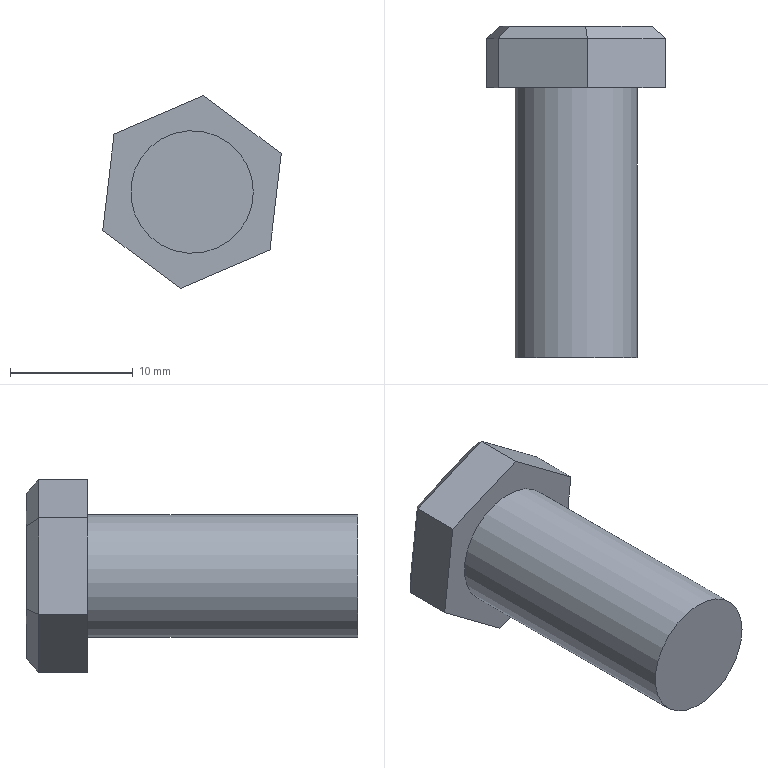Component | NX | LOC_PIN_2 | 1 solid | 16 faces | box 14.55 x 27 x 15.73 mm | volume 2520 mm3 | plane 15 | cylinder 1 | commonest cylinder face diameters 10 x1
STEP:
#1=CARTESIAN_POINT('',(0.,0.,0.));
#2=DIRECTION('',(0.,0.,1.));
#3=DIRECTION('',(1.,0.,0.));
#4=AXIS2_PLACEMENT_3D('',#1,#2,#3);
#5=CARTESIAN_POINT('',(68.825,100.796,50.));
#6=VERTEX_POINT('',#5);
#7=CARTESIAN_POINT('',(63.825,100.796,50.));
#8=DIRECTION('',(0.,-1.,0.));
#9=DIRECTION('',(1.,0.,0.));
#10=AXIS2_PLACEMENT_3D('',#7,#8,#9);
#11=CIRCLE('',#10,5.);
#12=CARTESIAN_POINT('',(63.825,100.796,50.));
#13=DIRECTION('',(0.,-1.,0.));
#14=DIRECTION('',(-1.,0.,0.));
#15=AXIS2_PLACEMENT_3D('',#12,#13,#14);
#16=CYLINDRICAL_SURFACE('',#15,5.);
#17=CARTESIAN_POINT('',(3.142,0.));
#18=DIRECTION('',(1.,0.));
#19=VECTOR('',#18,1.);
#20=LINE('',#17,#19);
#21=(GEOMETRIC_REPRESENTATION_CONTEXT(2)PARAMETRIC_REPRESENTATION_CONTEXT()REPRESENTATION_CONTEXT('',''));
#22=DEFINITIONAL_REPRESENTATION('',(#20),#21);
#23=PCURVE('',#16,#22);
#24=CARTESIAN_POINT('',(63.825,100.796,50.));
#25=DIRECTION('',(0.,-1.,0.));
#26=DIRECTION('',(-1.,0.,0.));
#27=AXIS2_PLACEMENT_3D('',#24,#25,#26);
#28=PLANE('',#27);
#29=CARTESIAN_POINT('',(0.,0.));
#30=DIRECTION('',(-1.,0.));
#31=AXIS2_PLACEMENT_2D('',#29,#30);
#32=CIRCLE('',#31,5.);
#33=(GEOMETRIC_REPRESENTATION_CONTEXT(2)PARAMETRIC_REPRESENTATION_CONTEXT()REPRESENTATION_CONTEXT('',''));
#34=DEFINITIONAL_REPRESENTATION('',(#32),#33);
#35=PCURVE('',#28,#34);
#36=SURFACE_CURVE('',#11,(#23,#35),.PCURVE_S1.);
#37=EDGE_CURVE('',#6,#6,#36,.T.);
#38=ORIENTED_EDGE('',*,*,#37,.T.);
#39=CARTESIAN_POINT('',(68.825,78.796,50.));
#40=VERTEX_POINT('',#39);
#41=CARTESIAN_POINT('',(68.825,100.796,50.));
#42=CARTESIAN_POINT('',(68.825,78.796,50.));
#43=B_SPLINE_CURVE_WITH_KNOTS('',1,(#41,#42),.UNSPECIFIED.,.F.,.F.,(2,2),(0.,22.),.PIECEWISE_BEZIER_KNOTS.);
#44=CARTESIAN_POINT('',(9.425,0.));
#45=DIRECTION('',(0.,1.));
#46=VECTOR('',#45,1.);
#47=LINE('',#44,#46);
#48=(GEOMETRIC_REPRESENTATION_CONTEXT(2)PARAMETRIC_REPRESENTATION_CONTEXT()REPRESENTATION_CONTEXT('',''));
#49=DEFINITIONAL_REPRESENTATION('',(#47),#48);
#50=PCURVE('',#16,#49);
#51=CARTESIAN_POINT('',(3.142,0.));
#52=DIRECTION('',(0.,1.));
#53=VECTOR('',#52,1.);
#54=LINE('',#51,#53);
#55=(GEOMETRIC_REPRESENTATION_CONTEXT(2)PARAMETRIC_REPRESENTATION_CONTEXT()REPRESENTATION_CONTEXT('',''));
#56=DEFINITIONAL_REPRESENTATION('',(#54),#55);
#57=PCURVE('',#16,#56);
#58=SEAM_CURVE('',#43,(#50,#57),.PCURVE_S1.);
#59=EDGE_CURVE('',#6,#40,#58,.T.);
#60=ORIENTED_EDGE('',*,*,#59,.T.);
#61=CARTESIAN_POINT('',(63.825,78.796,50.));
#62=DIRECTION('',(0.,-1.,0.));
#63=DIRECTION('',(1.,0.,0.));
#64=AXIS2_PLACEMENT_3D('',#61,#62,#63);
#65=CIRCLE('',#64,5.);
#66=CARTESIAN_POINT('',(3.142,22.));
#67=DIRECTION('',(1.,0.));
#68=VECTOR('',#67,1.);
#69=LINE('',#66,#68);
#70=(GEOMETRIC_REPRESENTATION_CONTEXT(2)PARAMETRIC_REPRESENTATION_CONTEXT()REPRESENTATION_CONTEXT('',''));
#71=DEFINITIONAL_REPRESENTATION('',(#69),#70);
#72=PCURVE('',#16,#71);
#73=CARTESIAN_POINT('',(63.825,78.796,50.));
#74=DIRECTION('',(0.,-1.,0.));
#75=DIRECTION('',(-1.,0.,0.));
#76=AXIS2_PLACEMENT_3D('',#73,#74,#75);
#77=PLANE('',#76);
#78=CARTESIAN_POINT('',(0.,0.));
#79=DIRECTION('',(-1.,0.));
#80=AXIS2_PLACEMENT_2D('',#78,#79);
#81=CIRCLE('',#80,5.);
#82=(GEOMETRIC_REPRESENTATION_CONTEXT(2)PARAMETRIC_REPRESENTATION_CONTEXT()REPRESENTATION_CONTEXT('',''));
#83=DEFINITIONAL_REPRESENTATION('',(#81),#82);
#84=PCURVE('',#77,#83);
#85=SURFACE_CURVE('',#65,(#72,#84),.PCURVE_S1.);
#86=EDGE_CURVE('',#40,#40,#85,.T.);
#87=ORIENTED_EDGE('',*,*,#86,.F.);
#88=ORIENTED_EDGE('',*,*,#59,.F.);
#89=EDGE_LOOP('',(#38,#60,#87,#88));
#90=FACE_BOUND('',#89,.T.);
#91=ADVANCED_FACE('',(#90),#16,.T.);
#92=ORIENTED_EDGE('',*,*,#86,.T.);
#93=EDGE_LOOP('',(#92));
#94=FACE_BOUND('',#93,.T.);
#95=ADVANCED_FACE('',(#94),#77,.T.);
#96=CARTESIAN_POINT('',(56.548,104.796,46.869));
#97=VERTEX_POINT('',#96);
#98=CARTESIAN_POINT('',(56.548,100.796,46.869));
#99=VERTEX_POINT('',#98);
#100=CARTESIAN_POINT('',(56.548,105.796,46.869));
#101=DIRECTION('',(0.,-1.,0.));
#102=VECTOR('',#101,1.);
#103=LINE('',#100,#102);
#104=CARTESIAN_POINT('',(56.548,105.796,46.869));
#105=DIRECTION('',(-0.5979,0.,-0.8016));
#106=DIRECTION('',(-0.8016,0.,0.5979));
#107=AXIS2_PLACEMENT_3D('',#104,#105,#106);
#108=PLANE('',#107);
#109=CARTESIAN_POINT('',(0.,0.));
#110=DIRECTION('',(0.,-1.));
#111=VECTOR('',#110,1.);
#112=LINE('',#109,#111);
#113=(GEOMETRIC_REPRESENTATION_CONTEXT(2)PARAMETRIC_REPRESENTATION_CONTEXT()REPRESENTATION_CONTEXT('',''));
#114=DEFINITIONAL_REPRESENTATION('',(#112),#113);
#115=PCURVE('',#108,#114);
#116=CARTESIAN_POINT('',(57.475,105.796,54.736));
#117=DIRECTION('',(-0.9931,0.,0.117));
#118=DIRECTION('',(0.117,0.,0.9931));
#119=AXIS2_PLACEMENT_3D('',#116,#117,#118);
#120=PLANE('',#119);
#121=CARTESIAN_POINT('',(-7.922,0.));
#122=DIRECTION('',(0.,-1.));
#123=VECTOR('',#122,1.);
#124=LINE('',#121,#123);
#125=(GEOMETRIC_REPRESENTATION_CONTEXT(2)PARAMETRIC_REPRESENTATION_CONTEXT()REPRESENTATION_CONTEXT('',''));
#126=DEFINITIONAL_REPRESENTATION('',(#124),#125);
#127=PCURVE('',#120,#126);
#128=SURFACE_CURVE('',#103,(#115,#127),.PCURVE_S1.);
#129=EDGE_CURVE('',#97,#99,#128,.T.);
#130=ORIENTED_EDGE('',*,*,#129,.F.);
#131=CARTESIAN_POINT('',(62.898,104.796,42.133));
#132=VERTEX_POINT('',#131);
#133=CARTESIAN_POINT('',(62.898,104.796,42.133));
#134=DIRECTION('',(0.8016,0.,-0.5979));
#135=VECTOR('',#134,1.);
#136=LINE('',#133,#135);
#137=CARTESIAN_POINT('',(-7.922,-1.));
#138=DIRECTION('',(-1.,0.));
#139=VECTOR('',#138,1.);
#140=LINE('',#137,#139);
#141=(GEOMETRIC_REPRESENTATION_CONTEXT(2)PARAMETRIC_REPRESENTATION_CONTEXT()REPRESENTATION_CONTEXT('',''));
#142=DEFINITIONAL_REPRESENTATION('',(#140),#141);
#143=PCURVE('',#108,#142);
#144=CARTESIAN_POINT('',(56.548,104.796,46.869));
#145=DIRECTION('',(-0.4228,0.7071,-0.5668));
#146=DIRECTION('',(-0.8016,0.,0.5979));
#147=AXIS2_PLACEMENT_3D('',#144,#145,#146);
#148=PLANE('',#147);
#149=CARTESIAN_POINT('',(-7.922,-0.));
#150=DIRECTION('',(-1.,0.));
#151=VECTOR('',#150,1.);
#152=LINE('',#149,#151);
#153=(GEOMETRIC_REPRESENTATION_CONTEXT(2)PARAMETRIC_REPRESENTATION_CONTEXT()REPRESENTATION_CONTEXT('',''));
#154=DEFINITIONAL_REPRESENTATION('',(#152),#153);
#155=PCURVE('',#148,#154);
#156=SURFACE_CURVE('',#136,(#143,#155),.PCURVE_S1.);
#157=EDGE_CURVE('',#97,#132,#156,.T.);
#158=ORIENTED_EDGE('',*,*,#157,.T.);
#159=CARTESIAN_POINT('',(62.898,100.796,42.133));
#160=VERTEX_POINT('',#159);
#161=CARTESIAN_POINT('',(62.898,105.796,42.133));
#162=DIRECTION('',(0.,-1.,0.));
#163=VECTOR('',#162,1.);
#164=LINE('',#161,#163);
#165=CARTESIAN_POINT('',(-7.922,0.));
#166=DIRECTION('',(0.,-1.));
#167=VECTOR('',#166,1.);
#168=LINE('',#165,#167);
#169=(GEOMETRIC_REPRESENTATION_CONTEXT(2)PARAMETRIC_REPRESENTATION_CONTEXT()REPRESENTATION_CONTEXT('',''));
#170=DEFINITIONAL_REPRESENTATION('',(#168),#169);
#171=PCURVE('',#108,#170);
#172=CARTESIAN_POINT('',(62.898,105.796,42.133));
#173=DIRECTION('',(0.3953,0.,-0.9186));
#174=DIRECTION('',(-0.9186,0.,-0.3953));
#175=AXIS2_PLACEMENT_3D('',#172,#173,#174);
#176=PLANE('',#175);
#177=CARTESIAN_POINT('',(0.,0.));
#178=DIRECTION('',(0.,-1.));
#179=VECTOR('',#178,1.);
#180=LINE('',#177,#179);
#181=(GEOMETRIC_REPRESENTATION_CONTEXT(2)PARAMETRIC_REPRESENTATION_CONTEXT()REPRESENTATION_CONTEXT('',''));
#182=DEFINITIONAL_REPRESENTATION('',(#180),#181);
#183=PCURVE('',#176,#182);
#184=SURFACE_CURVE('',#164,(#171,#183),.PCURVE_S1.);
#185=EDGE_CURVE('',#132,#160,#184,.T.);
#186=ORIENTED_EDGE('',*,*,#185,.T.);
#187=CARTESIAN_POINT('',(56.548,100.796,46.869));
#188=DIRECTION('',(0.8016,0.,-0.5979));
#189=VECTOR('',#188,1.);
#190=LINE('',#187,#189);
#191=CARTESIAN_POINT('',(0.,-5.));
#192=DIRECTION('',(-1.,0.));
#193=VECTOR('',#192,1.);
#194=LINE('',#191,#193);
#195=(GEOMETRIC_REPRESENTATION_CONTEXT(2)PARAMETRIC_REPRESENTATION_CONTEXT()REPRESENTATION_CONTEXT('',''));
#196=DEFINITIONAL_REPRESENTATION('',(#194),#195);
#197=PCURVE('',#108,#196);
#198=CARTESIAN_POINT('',(7.277,3.131));
#199=DIRECTION('',(-0.8016,0.5979));
#200=VECTOR('',#199,1.);
#201=LINE('',#198,#200);
#202=(GEOMETRIC_REPRESENTATION_CONTEXT(2)PARAMETRIC_REPRESENTATION_CONTEXT()REPRESENTATION_CONTEXT('',''));
#203=DEFINITIONAL_REPRESENTATION('',(#201),#202);
#204=PCURVE('',#28,#203);
#205=SURFACE_CURVE('',#190,(#197,#204),.PCURVE_S1.);
#206=EDGE_CURVE('',#99,#160,#205,.T.);
#207=ORIENTED_EDGE('',*,*,#206,.F.);
#208=EDGE_LOOP('',(#130,#158,#186,#207));
#209=FACE_BOUND('',#208,.T.);
#210=ADVANCED_FACE('',(#209),#108,.T.);
#211=ORIENTED_EDGE('',*,*,#185,.F.);
#212=CARTESIAN_POINT('',(70.175,104.796,45.264));
#213=VERTEX_POINT('',#212);
#214=CARTESIAN_POINT('',(70.175,104.796,45.264));
#215=DIRECTION('',(0.9186,0.,0.3953));
#216=VECTOR('',#215,1.);
#217=LINE('',#214,#216);
#218=CARTESIAN_POINT('',(-7.922,-1.));
#219=DIRECTION('',(-1.,0.));
#220=VECTOR('',#219,1.);
#221=LINE('',#218,#220);
#222=(GEOMETRIC_REPRESENTATION_CONTEXT(2)PARAMETRIC_REPRESENTATION_CONTEXT()REPRESENTATION_CONTEXT('',''));
#223=DEFINITIONAL_REPRESENTATION('',(#221),#222);
#224=PCURVE('',#176,#223);
#225=CARTESIAN_POINT('',(62.898,104.796,42.133));
#226=DIRECTION('',(0.2795,0.7071,-0.6495));
#227=DIRECTION('',(-0.9186,0.,-0.3953));
#228=AXIS2_PLACEMENT_3D('',#225,#226,#227);
#229=PLANE('',#228);
#230=CARTESIAN_POINT('',(-7.922,-0.));
#231=DIRECTION('',(-1.,0.));
#232=VECTOR('',#231,1.);
#233=LINE('',#230,#232);
#234=(GEOMETRIC_REPRESENTATION_CONTEXT(2)PARAMETRIC_REPRESENTATION_CONTEXT()REPRESENTATION_CONTEXT('',''));
#235=DEFINITIONAL_REPRESENTATION('',(#233),#234);
#236=PCURVE('',#229,#235);
#237=SURFACE_CURVE('',#217,(#224,#236),.PCURVE_S1.);
#238=EDGE_CURVE('',#132,#213,#237,.T.);
#239=ORIENTED_EDGE('',*,*,#238,.T.);
#240=CARTESIAN_POINT('',(70.175,100.796,45.264));
#241=VERTEX_POINT('',#240);
#242=CARTESIAN_POINT('',(70.175,105.796,45.264));
#243=DIRECTION('',(0.,-1.,0.));
#244=VECTOR('',#243,1.);
#245=LINE('',#242,#244);
#246=CARTESIAN_POINT('',(-7.922,0.));
#247=DIRECTION('',(0.,-1.));
#248=VECTOR('',#247,1.);
#249=LINE('',#246,#248);
#250=(GEOMETRIC_REPRESENTATION_CONTEXT(2)PARAMETRIC_REPRESENTATION_CONTEXT()REPRESENTATION_CONTEXT('',''));
#251=DEFINITIONAL_REPRESENTATION('',(#249),#250);
#252=PCURVE('',#176,#251);
#253=CARTESIAN_POINT('',(70.175,105.796,45.264));
#254=DIRECTION('',(0.9931,0.,-0.117));
#255=DIRECTION('',(-0.117,0.,-0.9931));
#256=AXIS2_PLACEMENT_3D('',#253,#254,#255);
#257=PLANE('',#256);
#258=CARTESIAN_POINT('',(0.,0.));
#259=DIRECTION('',(0.,-1.));
#260=VECTOR('',#259,1.);
#261=LINE('',#258,#260);
#262=(GEOMETRIC_REPRESENTATION_CONTEXT(2)PARAMETRIC_REPRESENTATION_CONTEXT()REPRESENTATION_CONTEXT('',''));
#263=DEFINITIONAL_REPRESENTATION('',(#261),#262);
#264=PCURVE('',#257,#263);
#265=SURFACE_CURVE('',#245,(#252,#264),.PCURVE_S1.);
#266=EDGE_CURVE('',#213,#241,#265,.T.);
#267=ORIENTED_EDGE('',*,*,#266,.T.);
#268=CARTESIAN_POINT('',(62.898,100.796,42.133));
#269=DIRECTION('',(0.9186,0.,0.3953));
#270=VECTOR('',#269,1.);
#271=LINE('',#268,#270);
#272=CARTESIAN_POINT('',(0.,-5.));
#273=DIRECTION('',(-1.,0.));
#274=VECTOR('',#273,1.);
#275=LINE('',#272,#274);
#276=(GEOMETRIC_REPRESENTATION_CONTEXT(2)PARAMETRIC_REPRESENTATION_CONTEXT()REPRESENTATION_CONTEXT('',''));
#277=DEFINITIONAL_REPRESENTATION('',(#275),#276);
#278=PCURVE('',#176,#277);
#279=CARTESIAN_POINT('',(0.9266,7.867));
#280=DIRECTION('',(-0.9186,-0.3953));
#281=VECTOR('',#280,1.);
#282=LINE('',#279,#281);
#283=(GEOMETRIC_REPRESENTATION_CONTEXT(2)PARAMETRIC_REPRESENTATION_CONTEXT()REPRESENTATION_CONTEXT('',''));
#284=DEFINITIONAL_REPRESENTATION('',(#282),#283);
#285=PCURVE('',#28,#284);
#286=SURFACE_CURVE('',#271,(#278,#285),.PCURVE_S1.);
#287=EDGE_CURVE('',#160,#241,#286,.T.);
#288=ORIENTED_EDGE('',*,*,#287,.F.);
#289=EDGE_LOOP('',(#211,#239,#267,#288));
#290=FACE_BOUND('',#289,.T.);
#291=ADVANCED_FACE('',(#290),#176,.T.);
#292=ORIENTED_EDGE('',*,*,#266,.F.);
#293=CARTESIAN_POINT('',(71.101,104.796,53.131));
#294=VERTEX_POINT('',#293);
#295=CARTESIAN_POINT('',(71.101,104.796,53.131));
#296=DIRECTION('',(0.117,0.,0.9931));
#297=VECTOR('',#296,1.);
#298=LINE('',#295,#297);
#299=CARTESIAN_POINT('',(-7.922,-1.));
#300=DIRECTION('',(-1.,0.));
#301=VECTOR('',#300,1.);
#302=LINE('',#299,#301);
#303=(GEOMETRIC_REPRESENTATION_CONTEXT(2)PARAMETRIC_REPRESENTATION_CONTEXT()REPRESENTATION_CONTEXT('',''));
#304=DEFINITIONAL_REPRESENTATION('',(#302),#303);
#305=PCURVE('',#257,#304);
#306=CARTESIAN_POINT('',(70.175,104.796,45.264));
#307=DIRECTION('',(0.7023,0.7071,-0.08271));
#308=DIRECTION('',(-0.117,0.,-0.9931));
#309=AXIS2_PLACEMENT_3D('',#306,#307,#308);
#310=PLANE('',#309);
#311=CARTESIAN_POINT('',(-7.922,-0.));
#312=DIRECTION('',(-1.,0.));
#313=VECTOR('',#312,1.);
#314=LINE('',#311,#313);
#315=(GEOMETRIC_REPRESENTATION_CONTEXT(2)PARAMETRIC_REPRESENTATION_CONTEXT()REPRESENTATION_CONTEXT('',''));
#316=DEFINITIONAL_REPRESENTATION('',(#314),#315);
#317=PCURVE('',#310,#316);
#318=SURFACE_CURVE('',#298,(#305,#317),.PCURVE_S1.);
#319=EDGE_CURVE('',#213,#294,#318,.T.);
#320=ORIENTED_EDGE('',*,*,#319,.T.);
#321=CARTESIAN_POINT('',(71.101,100.796,53.131));
#322=VERTEX_POINT('',#321);
#323=CARTESIAN_POINT('',(71.101,105.796,53.131));
#324=DIRECTION('',(0.,-1.,0.));
#325=VECTOR('',#324,1.);
#326=LINE('',#323,#325);
#327=CARTESIAN_POINT('',(-7.922,0.));
#328=DIRECTION('',(0.,-1.));
#329=VECTOR('',#328,1.);
#330=LINE('',#327,#329);
#331=(GEOMETRIC_REPRESENTATION_CONTEXT(2)PARAMETRIC_REPRESENTATION_CONTEXT()REPRESENTATION_CONTEXT('',''));
#332=DEFINITIONAL_REPRESENTATION('',(#330),#331);
#333=PCURVE('',#257,#332);
#334=CARTESIAN_POINT('',(71.101,105.796,53.131));
#335=DIRECTION('',(0.5979,0.,0.8016));
#336=DIRECTION('',(0.8016,0.,-0.5979));
#337=AXIS2_PLACEMENT_3D('',#334,#335,#336);
#338=PLANE('',#337);
#339=CARTESIAN_POINT('',(0.,0.));
#340=DIRECTION('',(0.,-1.));
#341=VECTOR('',#340,1.);
#342=LINE('',#339,#341);
#343=(GEOMETRIC_REPRESENTATION_CONTEXT(2)PARAMETRIC_REPRESENTATION_CONTEXT()REPRESENTATION_CONTEXT('',''));
#344=DEFINITIONAL_REPRESENTATION('',(#342),#343);
#345=PCURVE('',#338,#344);
#346=SURFACE_CURVE('',#326,(#333,#345),.PCURVE_S1.);
#347=EDGE_CURVE('',#294,#322,#346,.T.);
#348=ORIENTED_EDGE('',*,*,#347,.T.);
#349=CARTESIAN_POINT('',(70.175,100.796,45.264));
#350=DIRECTION('',(0.117,0.,0.9931));
#351=VECTOR('',#350,1.);
#352=LINE('',#349,#351);
#353=CARTESIAN_POINT('',(0.,-5.));
#354=DIRECTION('',(-1.,0.));
#355=VECTOR('',#354,1.);
#356=LINE('',#353,#355);
#357=(GEOMETRIC_REPRESENTATION_CONTEXT(2)PARAMETRIC_REPRESENTATION_CONTEXT()REPRESENTATION_CONTEXT('',''));
#358=DEFINITIONAL_REPRESENTATION('',(#356),#357);
#359=PCURVE('',#257,#358);
#360=CARTESIAN_POINT('',(-6.35,4.736));
#361=DIRECTION('',(-0.117,-0.9931));
#362=VECTOR('',#361,1.);
#363=LINE('',#360,#362);
#364=(GEOMETRIC_REPRESENTATION_CONTEXT(2)PARAMETRIC_REPRESENTATION_CONTEXT()REPRESENTATION_CONTEXT('',''));
#365=DEFINITIONAL_REPRESENTATION('',(#363),#364);
#366=PCURVE('',#28,#365);
#367=SURFACE_CURVE('',#352,(#359,#366),.PCURVE_S1.);
#368=EDGE_CURVE('',#241,#322,#367,.T.);
#369=ORIENTED_EDGE('',*,*,#368,.F.);
#370=EDGE_LOOP('',(#292,#320,#348,#369));
#371=FACE_BOUND('',#370,.T.);
#372=ADVANCED_FACE('',(#371),#257,.T.);
#373=ORIENTED_EDGE('',*,*,#347,.F.);
#374=CARTESIAN_POINT('',(64.751,104.796,57.867));
#375=VERTEX_POINT('',#374);
#376=CARTESIAN_POINT('',(64.751,104.796,57.867));
#377=DIRECTION('',(-0.8016,0.,0.5979));
#378=VECTOR('',#377,1.);
#379=LINE('',#376,#378);
#380=CARTESIAN_POINT('',(-7.922,-1.));
#381=DIRECTION('',(-1.,0.));
#382=VECTOR('',#381,1.);
#383=LINE('',#380,#382);
#384=(GEOMETRIC_REPRESENTATION_CONTEXT(2)PARAMETRIC_REPRESENTATION_CONTEXT()REPRESENTATION_CONTEXT('',''));
#385=DEFINITIONAL_REPRESENTATION('',(#383),#384);
#386=PCURVE('',#338,#385);
#387=CARTESIAN_POINT('',(71.101,104.796,53.131));
#388=DIRECTION('',(0.4228,0.7071,0.5668));
#389=DIRECTION('',(0.8016,0.,-0.5979));
#390=AXIS2_PLACEMENT_3D('',#387,#388,#389);
#391=PLANE('',#390);
#392=CARTESIAN_POINT('',(-7.922,0.));
#393=DIRECTION('',(-1.,0.));
#394=VECTOR('',#393,1.);
#395=LINE('',#392,#394);
#396=(GEOMETRIC_REPRESENTATION_CONTEXT(2)PARAMETRIC_REPRESENTATION_CONTEXT()REPRESENTATION_CONTEXT('',''));
#397=DEFINITIONAL_REPRESENTATION('',(#395),#396);
#398=PCURVE('',#391,#397);
#399=SURFACE_CURVE('',#379,(#386,#398),.PCURVE_S1.);
#400=EDGE_CURVE('',#294,#375,#399,.T.);
#401=ORIENTED_EDGE('',*,*,#400,.T.);
#402=CARTESIAN_POINT('',(64.751,100.796,57.867));
#403=VERTEX_POINT('',#402);
#404=CARTESIAN_POINT('',(64.751,105.796,57.867));
#405=DIRECTION('',(0.,-1.,0.));
#406=VECTOR('',#405,1.);
#407=LINE('',#404,#406);
#408=CARTESIAN_POINT('',(-7.922,0.));
#409=DIRECTION('',(0.,-1.));
#410=VECTOR('',#409,1.);
#411=LINE('',#408,#410);
#412=(GEOMETRIC_REPRESENTATION_CONTEXT(2)PARAMETRIC_REPRESENTATION_CONTEXT()REPRESENTATION_CONTEXT('',''));
#413=DEFINITIONAL_REPRESENTATION('',(#411),#412);
#414=PCURVE('',#338,#413);
#415=CARTESIAN_POINT('',(64.751,105.796,57.867));
#416=DIRECTION('',(-0.3953,0.,0.9186));
#417=DIRECTION('',(0.9186,0.,0.3953));
#418=AXIS2_PLACEMENT_3D('',#415,#416,#417);
#419=PLANE('',#418);
#420=CARTESIAN_POINT('',(0.,0.));
#421=DIRECTION('',(0.,-1.));
#422=VECTOR('',#421,1.);
#423=LINE('',#420,#422);
#424=(GEOMETRIC_REPRESENTATION_CONTEXT(2)PARAMETRIC_REPRESENTATION_CONTEXT()REPRESENTATION_CONTEXT('',''));
#425=DEFINITIONAL_REPRESENTATION('',(#423),#424);
#426=PCURVE('',#419,#425);
#427=SURFACE_CURVE('',#407,(#414,#426),.PCURVE_S1.);
#428=EDGE_CURVE('',#375,#403,#427,.T.);
#429=ORIENTED_EDGE('',*,*,#428,.T.);
#430=CARTESIAN_POINT('',(71.101,100.796,53.131));
#431=DIRECTION('',(-0.8016,0.,0.5979));
#432=VECTOR('',#431,1.);
#433=LINE('',#430,#432);
#434=CARTESIAN_POINT('',(0.,-5.));
#435=DIRECTION('',(-1.,0.));
#436=VECTOR('',#435,1.);
#437=LINE('',#434,#436);
#438=(GEOMETRIC_REPRESENTATION_CONTEXT(2)PARAMETRIC_REPRESENTATION_CONTEXT()REPRESENTATION_CONTEXT('',''));
#439=DEFINITIONAL_REPRESENTATION('',(#437),#438);
#440=PCURVE('',#338,#439);
#441=CARTESIAN_POINT('',(-7.277,-3.131));
#442=DIRECTION('',(0.8016,-0.5979));
#443=VECTOR('',#442,1.);
#444=LINE('',#441,#443);
#445=(GEOMETRIC_REPRESENTATION_CONTEXT(2)PARAMETRIC_REPRESENTATION_CONTEXT()REPRESENTATION_CONTEXT('',''));
#446=DEFINITIONAL_REPRESENTATION('',(#444),#445);
#447=PCURVE('',#28,#446);
#448=SURFACE_CURVE('',#433,(#440,#447),.PCURVE_S1.);
#449=EDGE_CURVE('',#322,#403,#448,.T.);
#450=ORIENTED_EDGE('',*,*,#449,.F.);
#451=EDGE_LOOP('',(#373,#401,#429,#450));
#452=FACE_BOUND('',#451,.T.);
#453=ADVANCED_FACE('',(#452),#338,.T.);
#454=ORIENTED_EDGE('',*,*,#428,.F.);
#455=CARTESIAN_POINT('',(57.475,104.796,54.736));
#456=VERTEX_POINT('',#455);
#457=CARTESIAN_POINT('',(57.475,104.796,54.736));
#458=DIRECTION('',(-0.9186,0.,-0.3953));
#459=VECTOR('',#458,1.);
#460=LINE('',#457,#459);
#461=CARTESIAN_POINT('',(-7.922,-1.));
#462=DIRECTION('',(-1.,0.));
#463=VECTOR('',#462,1.);
#464=LINE('',#461,#463);
#465=(GEOMETRIC_REPRESENTATION_CONTEXT(2)PARAMETRIC_REPRESENTATION_CONTEXT()REPRESENTATION_CONTEXT('',''));
#466=DEFINITIONAL_REPRESENTATION('',(#464),#465);
#467=PCURVE('',#419,#466);
#468=CARTESIAN_POINT('',(64.751,104.796,57.867));
#469=DIRECTION('',(-0.2795,0.7071,0.6495));
#470=DIRECTION('',(0.9186,-0.,0.3953));
#471=AXIS2_PLACEMENT_3D('',#468,#469,#470);
#472=PLANE('',#471);
#473=CARTESIAN_POINT('',(-7.922,0.));
#474=DIRECTION('',(-1.,0.));
#475=VECTOR('',#474,1.);
#476=LINE('',#473,#475);
#477=(GEOMETRIC_REPRESENTATION_CONTEXT(2)PARAMETRIC_REPRESENTATION_CONTEXT()REPRESENTATION_CONTEXT('',''));
#478=DEFINITIONAL_REPRESENTATION('',(#476),#477);
#479=PCURVE('',#472,#478);
#480=SURFACE_CURVE('',#460,(#467,#479),.PCURVE_S1.);
#481=EDGE_CURVE('',#375,#456,#480,.T.);
#482=ORIENTED_EDGE('',*,*,#481,.T.);
#483=CARTESIAN_POINT('',(57.475,100.796,54.736));
#484=VERTEX_POINT('',#483);
#485=CARTESIAN_POINT('',(57.475,105.796,54.736));
#486=DIRECTION('',(0.,-1.,0.));
#487=VECTOR('',#486,1.);
#488=LINE('',#485,#487);
#489=CARTESIAN_POINT('',(-7.922,0.));
#490=DIRECTION('',(0.,-1.));
#491=VECTOR('',#490,1.);
#492=LINE('',#489,#491);
#493=(GEOMETRIC_REPRESENTATION_CONTEXT(2)PARAMETRIC_REPRESENTATION_CONTEXT()REPRESENTATION_CONTEXT('',''));
#494=DEFINITIONAL_REPRESENTATION('',(#492),#493);
#495=PCURVE('',#419,#494);
#496=CARTESIAN_POINT('',(0.,0.));
#497=DIRECTION('',(0.,-1.));
#498=VECTOR('',#497,1.);
#499=LINE('',#496,#498);
#500=(GEOMETRIC_REPRESENTATION_CONTEXT(2)PARAMETRIC_REPRESENTATION_CONTEXT()REPRESENTATION_CONTEXT('',''));
#501=DEFINITIONAL_REPRESENTATION('',(#499),#500);
#502=PCURVE('',#120,#501);
#503=SURFACE_CURVE('',#488,(#495,#502),.PCURVE_S1.);
#504=EDGE_CURVE('',#456,#484,#503,.T.);
#505=ORIENTED_EDGE('',*,*,#504,.T.);
#506=CARTESIAN_POINT('',(64.751,100.796,57.867));
#507=DIRECTION('',(-0.9186,0.,-0.3953));
#508=VECTOR('',#507,1.);
#509=LINE('',#506,#508);
#510=CARTESIAN_POINT('',(0.,-5.));
#511=DIRECTION('',(-1.,0.));
#512=VECTOR('',#511,1.);
#513=LINE('',#510,#512);
#514=(GEOMETRIC_REPRESENTATION_CONTEXT(2)PARAMETRIC_REPRESENTATION_CONTEXT()REPRESENTATION_CONTEXT('',''));
#515=DEFINITIONAL_REPRESENTATION('',(#513),#514);
#516=PCURVE('',#419,#515);
#517=CARTESIAN_POINT('',(-0.9266,-7.867));
#518=DIRECTION('',(0.9186,0.3953));
#519=VECTOR('',#518,1.);
#520=LINE('',#517,#519);
#521=(GEOMETRIC_REPRESENTATION_CONTEXT(2)PARAMETRIC_REPRESENTATION_CONTEXT()REPRESENTATION_CONTEXT('',''));
#522=DEFINITIONAL_REPRESENTATION('',(#520),#521);
#523=PCURVE('',#28,#522);
#524=SURFACE_CURVE('',#509,(#516,#523),.PCURVE_S1.);
#525=EDGE_CURVE('',#403,#484,#524,.T.);
#526=ORIENTED_EDGE('',*,*,#525,.F.);
#527=EDGE_LOOP('',(#454,#482,#505,#526));
#528=FACE_BOUND('',#527,.T.);
#529=ADVANCED_FACE('',(#528),#419,.T.);
#530=ORIENTED_EDGE('',*,*,#504,.F.);
#531=CARTESIAN_POINT('',(56.548,104.796,46.869));
#532=DIRECTION('',(-0.117,0.,-0.9931));
#533=VECTOR('',#532,1.);
#534=LINE('',#531,#533);
#535=CARTESIAN_POINT('',(-7.922,-1.));
#536=DIRECTION('',(-1.,0.));
#537=VECTOR('',#536,1.);
#538=LINE('',#535,#537);
#539=(GEOMETRIC_REPRESENTATION_CONTEXT(2)PARAMETRIC_REPRESENTATION_CONTEXT()REPRESENTATION_CONTEXT('',''));
#540=DEFINITIONAL_REPRESENTATION('',(#538),#539);
#541=PCURVE('',#120,#540);
#542=CARTESIAN_POINT('',(57.475,104.796,54.736));
#543=DIRECTION('',(-0.7023,0.7071,0.08271));
#544=DIRECTION('',(0.117,-0.,0.9931));
#545=AXIS2_PLACEMENT_3D('',#542,#543,#544);
#546=PLANE('',#545);
#547=CARTESIAN_POINT('',(-7.922,0.));
#548=DIRECTION('',(-1.,-0.));
#549=VECTOR('',#548,1.);
#550=LINE('',#547,#549);
#551=(GEOMETRIC_REPRESENTATION_CONTEXT(2)PARAMETRIC_REPRESENTATION_CONTEXT()REPRESENTATION_CONTEXT('',''));
#552=DEFINITIONAL_REPRESENTATION('',(#550),#551);
#553=PCURVE('',#546,#552);
#554=SURFACE_CURVE('',#534,(#541,#553),.PCURVE_S1.);
#555=EDGE_CURVE('',#456,#97,#554,.T.);
#556=ORIENTED_EDGE('',*,*,#555,.T.);
#557=ORIENTED_EDGE('',*,*,#129,.T.);
#558=CARTESIAN_POINT('',(57.475,100.796,54.736));
#559=DIRECTION('',(-0.117,0.,-0.9931));
#560=VECTOR('',#559,1.);
#561=LINE('',#558,#560);
#562=CARTESIAN_POINT('',(0.,-5.));
#563=DIRECTION('',(-1.,0.));
#564=VECTOR('',#563,1.);
#565=LINE('',#562,#564);
#566=(GEOMETRIC_REPRESENTATION_CONTEXT(2)PARAMETRIC_REPRESENTATION_CONTEXT()REPRESENTATION_CONTEXT('',''));
#567=DEFINITIONAL_REPRESENTATION('',(#565),#566);
#568=PCURVE('',#120,#567);
#569=CARTESIAN_POINT('',(6.35,-4.736));
#570=DIRECTION('',(0.117,0.9931));
#571=VECTOR('',#570,1.);
#572=LINE('',#569,#571);
#573=(GEOMETRIC_REPRESENTATION_CONTEXT(2)PARAMETRIC_REPRESENTATION_CONTEXT()REPRESENTATION_CONTEXT('',''));
#574=DEFINITIONAL_REPRESENTATION('',(#572),#573);
#575=PCURVE('',#28,#574);
#576=SURFACE_CURVE('',#561,(#568,#575),.PCURVE_S1.);
#577=EDGE_CURVE('',#484,#99,#576,.T.);
#578=ORIENTED_EDGE('',*,*,#577,.F.);
#579=EDGE_LOOP('',(#530,#556,#557,#578));
#580=FACE_BOUND('',#579,.T.);
#581=ADVANCED_FACE('',(#580),#120,.T.);
#582=CARTESIAN_POINT('',(63.033,105.796,43.279));
#583=VERTEX_POINT('',#582);
#584=CARTESIAN_POINT('',(57.609,105.796,47.325));
#585=VERTEX_POINT('',#584);
#586=CARTESIAN_POINT('',(57.146,105.796,47.67));
#587=DIRECTION('',(-0.8016,0.,0.5979));
#588=VECTOR('',#587,1.);
#589=LINE('',#586,#588);
#590=CARTESIAN_POINT('',(63.825,105.796,50.));
#591=DIRECTION('',(0.,-1.,0.));
#592=DIRECTION('',(-1.,0.,0.));
#593=AXIS2_PLACEMENT_3D('',#590,#591,#592);
#594=PLANE('',#593);
#595=CARTESIAN_POINT('',(6.679,2.33));
#596=DIRECTION('',(0.8016,-0.5979));
#597=VECTOR('',#596,1.);
#598=LINE('',#595,#597);
#599=(GEOMETRIC_REPRESENTATION_CONTEXT(2)PARAMETRIC_REPRESENTATION_CONTEXT()REPRESENTATION_CONTEXT('',''));
#600=DEFINITIONAL_REPRESENTATION('',(#598),#599);
#601=PCURVE('',#594,#600);
#602=CARTESIAN_POINT('',(0.,1.414));
#603=DIRECTION('',(1.,0.));
#604=VECTOR('',#603,1.);
#605=LINE('',#602,#604);
#606=(GEOMETRIC_REPRESENTATION_CONTEXT(2)PARAMETRIC_REPRESENTATION_CONTEXT()REPRESENTATION_CONTEXT('',''));
#607=DEFINITIONAL_REPRESENTATION('',(#605),#606);
#608=PCURVE('',#148,#607);
#609=SURFACE_CURVE('',#589,(#601,#608),.PCURVE_S1.);
#610=EDGE_CURVE('',#583,#585,#609,.T.);
#611=ORIENTED_EDGE('',*,*,#610,.T.);
#612=CARTESIAN_POINT('',(58.4,105.796,54.046));
#613=VERTEX_POINT('',#612);
#614=CARTESIAN_POINT('',(58.468,105.796,54.619));
#615=DIRECTION('',(0.117,0.,0.9931));
#616=VECTOR('',#615,1.);
#617=LINE('',#614,#616);
#618=CARTESIAN_POINT('',(5.357,-4.619));
#619=DIRECTION('',(-0.117,-0.9931));
#620=VECTOR('',#619,1.);
#621=LINE('',#618,#620);
#622=(GEOMETRIC_REPRESENTATION_CONTEXT(2)PARAMETRIC_REPRESENTATION_CONTEXT()REPRESENTATION_CONTEXT('',''));
#623=DEFINITIONAL_REPRESENTATION('',(#621),#622);
#624=PCURVE('',#594,#623);
#625=CARTESIAN_POINT('',(0.,1.414));
#626=DIRECTION('',(1.,0.));
#627=VECTOR('',#626,1.);
#628=LINE('',#625,#627);
#629=(GEOMETRIC_REPRESENTATION_CONTEXT(2)PARAMETRIC_REPRESENTATION_CONTEXT()REPRESENTATION_CONTEXT('',''));
#630=DEFINITIONAL_REPRESENTATION('',(#628),#629);
#631=PCURVE('',#546,#630);
#632=SURFACE_CURVE('',#617,(#624,#631),.PCURVE_S1.);
#633=EDGE_CURVE('',#585,#613,#632,.T.);
#634=ORIENTED_EDGE('',*,*,#633,.T.);
#635=CARTESIAN_POINT('',(64.616,105.796,56.721));
#636=VERTEX_POINT('',#635);
#637=CARTESIAN_POINT('',(65.147,105.796,56.949));
#638=DIRECTION('',(0.9186,0.,0.3953));
#639=VECTOR('',#638,1.);
#640=LINE('',#637,#639);
#641=CARTESIAN_POINT('',(-1.322,-6.949));
#642=DIRECTION('',(-0.9186,-0.3953));
#643=VECTOR('',#642,1.);
#644=LINE('',#641,#643);
#645=(GEOMETRIC_REPRESENTATION_CONTEXT(2)PARAMETRIC_REPRESENTATION_CONTEXT()REPRESENTATION_CONTEXT('',''));
#646=DEFINITIONAL_REPRESENTATION('',(#644),#645);
#647=PCURVE('',#594,#646);
#648=CARTESIAN_POINT('',(0.,1.414));
#649=DIRECTION('',(1.,-0.));
#650=VECTOR('',#649,1.);
#651=LINE('',#648,#650);
#652=(GEOMETRIC_REPRESENTATION_CONTEXT(2)PARAMETRIC_REPRESENTATION_CONTEXT()REPRESENTATION_CONTEXT('',''));
#653=DEFINITIONAL_REPRESENTATION('',(#651),#652);
#654=PCURVE('',#472,#653);
#655=SURFACE_CURVE('',#640,(#647,#654),.PCURVE_S1.);
#656=EDGE_CURVE('',#613,#636,#655,.T.);
#657=ORIENTED_EDGE('',*,*,#656,.T.);
#658=CARTESIAN_POINT('',(70.041,105.796,52.675));
#659=VERTEX_POINT('',#658);
#660=CARTESIAN_POINT('',(70.504,105.796,52.33));
#661=DIRECTION('',(0.8016,0.,-0.5979));
#662=VECTOR('',#661,1.);
#663=LINE('',#660,#662);
#664=CARTESIAN_POINT('',(-6.679,-2.33));
#665=DIRECTION('',(-0.8016,0.5979));
#666=VECTOR('',#665,1.);
#667=LINE('',#664,#666);
#668=(GEOMETRIC_REPRESENTATION_CONTEXT(2)PARAMETRIC_REPRESENTATION_CONTEXT()REPRESENTATION_CONTEXT('',''));
#669=DEFINITIONAL_REPRESENTATION('',(#667),#668);
#670=PCURVE('',#594,#669);
#671=CARTESIAN_POINT('',(-0.,1.414));
#672=DIRECTION('',(1.,0.));
#673=VECTOR('',#672,1.);
#674=LINE('',#671,#673);
#675=(GEOMETRIC_REPRESENTATION_CONTEXT(2)PARAMETRIC_REPRESENTATION_CONTEXT()REPRESENTATION_CONTEXT('',''));
#676=DEFINITIONAL_REPRESENTATION('',(#674),#675);
#677=PCURVE('',#391,#676);
#678=SURFACE_CURVE('',#663,(#670,#677),.PCURVE_S1.);
#679=EDGE_CURVE('',#636,#659,#678,.T.);
#680=ORIENTED_EDGE('',*,*,#679,.T.);
#681=CARTESIAN_POINT('',(69.249,105.796,45.954));
#682=VERTEX_POINT('',#681);
#683=CARTESIAN_POINT('',(69.182,105.796,45.381));
#684=DIRECTION('',(-0.117,0.,-0.9931));
#685=VECTOR('',#684,1.);
#686=LINE('',#683,#685);
#687=CARTESIAN_POINT('',(-5.357,4.619));
#688=DIRECTION('',(0.117,0.9931));
#689=VECTOR('',#688,1.);
#690=LINE('',#687,#689);
#691=(GEOMETRIC_REPRESENTATION_CONTEXT(2)PARAMETRIC_REPRESENTATION_CONTEXT()REPRESENTATION_CONTEXT('',''));
#692=DEFINITIONAL_REPRESENTATION('',(#690),#691);
#693=PCURVE('',#594,#692);
#694=CARTESIAN_POINT('',(0.,1.414));
#695=DIRECTION('',(1.,0.));
#696=VECTOR('',#695,1.);
#697=LINE('',#694,#696);
#698=(GEOMETRIC_REPRESENTATION_CONTEXT(2)PARAMETRIC_REPRESENTATION_CONTEXT()REPRESENTATION_CONTEXT('',''));
#699=DEFINITIONAL_REPRESENTATION('',(#697),#698);
#700=PCURVE('',#310,#699);
#701=SURFACE_CURVE('',#686,(#693,#700),.PCURVE_S1.);
#702=EDGE_CURVE('',#659,#682,#701,.T.);
#703=ORIENTED_EDGE('',*,*,#702,.T.);
#704=CARTESIAN_POINT('',(62.503,105.796,43.051));
#705=DIRECTION('',(-0.9186,0.,-0.3953));
#706=VECTOR('',#705,1.);
#707=LINE('',#704,#706);
#708=CARTESIAN_POINT('',(1.322,6.949));
#709=DIRECTION('',(0.9186,0.3953));
#710=VECTOR('',#709,1.);
#711=LINE('',#708,#710);
#712=(GEOMETRIC_REPRESENTATION_CONTEXT(2)PARAMETRIC_REPRESENTATION_CONTEXT()REPRESENTATION_CONTEXT('',''));
#713=DEFINITIONAL_REPRESENTATION('',(#711),#712);
#714=PCURVE('',#594,#713);
#715=CARTESIAN_POINT('',(-0.,1.414));
#716=DIRECTION('',(1.,-0.));
#717=VECTOR('',#716,1.);
#718=LINE('',#715,#717);
#719=(GEOMETRIC_REPRESENTATION_CONTEXT(2)PARAMETRIC_REPRESENTATION_CONTEXT()REPRESENTATION_CONTEXT('',''));
#720=DEFINITIONAL_REPRESENTATION('',(#718),#719);
#721=PCURVE('',#229,#720);
#722=SURFACE_CURVE('',#707,(#714,#721),.PCURVE_S1.);
#723=EDGE_CURVE('',#682,#583,#722,.T.);
#724=ORIENTED_EDGE('',*,*,#723,.T.);
#725=EDGE_LOOP('',(#611,#634,#657,#680,#703,#724));
#726=FACE_BOUND('',#725,.T.);
#727=ADVANCED_FACE('',(#726),#594,.F.);
#728=ORIENTED_EDGE('',*,*,#37,.F.);
#729=EDGE_LOOP('',(#728));
#730=FACE_BOUND('',#729,.T.);
#731=ORIENTED_EDGE('',*,*,#206,.T.);
#732=ORIENTED_EDGE('',*,*,#287,.T.);
#733=ORIENTED_EDGE('',*,*,#368,.T.);
#734=ORIENTED_EDGE('',*,*,#449,.T.);
#735=ORIENTED_EDGE('',*,*,#525,.T.);
#736=ORIENTED_EDGE('',*,*,#577,.T.);
#737=EDGE_LOOP('',(#731,#732,#733,#734,#735,#736));
#738=FACE_BOUND('',#737,.T.);
#739=ADVANCED_FACE('',(#730,#738),#28,.T.);
#740=CARTESIAN_POINT('',(70.175,104.796,45.264));
#741=DIRECTION('',(0.606,-0.6547,-0.4519));
#742=VECTOR('',#741,1.);
#743=LINE('',#740,#742);
#744=CARTESIAN_POINT('',(0.,0.));
#745=DIRECTION('',(0.378,-0.9258));
#746=VECTOR('',#745,1.);
#747=LINE('',#744,#746);
#748=(GEOMETRIC_REPRESENTATION_CONTEXT(2)PARAMETRIC_REPRESENTATION_CONTEXT()REPRESENTATION_CONTEXT('',''));
#749=DEFINITIONAL_REPRESENTATION('',(#747),#748);
#750=PCURVE('',#310,#749);
#751=CARTESIAN_POINT('',(-7.922,-0.));
#752=DIRECTION('',(-0.378,-0.9258));
#753=VECTOR('',#752,1.);
#754=LINE('',#751,#753);
#755=(GEOMETRIC_REPRESENTATION_CONTEXT(2)PARAMETRIC_REPRESENTATION_CONTEXT()REPRESENTATION_CONTEXT('',''));
#756=DEFINITIONAL_REPRESENTATION('',(#754),#755);
#757=PCURVE('',#229,#756);
#758=SURFACE_CURVE('',#743,(#750,#757),.PCURVE_S1.);
#759=EDGE_CURVE('',#682,#213,#758,.T.);
#760=ORIENTED_EDGE('',*,*,#759,.F.);
#761=ORIENTED_EDGE('',*,*,#702,.F.);
#762=CARTESIAN_POINT('',(71.101,104.796,53.131));
#763=DIRECTION('',(-0.6944,0.6547,-0.2988));
#764=VECTOR('',#763,1.);
#765=LINE('',#762,#764);
#766=CARTESIAN_POINT('',(-7.922,-0.));
#767=DIRECTION('',(0.378,0.9258));
#768=VECTOR('',#767,1.);
#769=LINE('',#766,#768);
#770=(GEOMETRIC_REPRESENTATION_CONTEXT(2)PARAMETRIC_REPRESENTATION_CONTEXT()REPRESENTATION_CONTEXT('',''));
#771=DEFINITIONAL_REPRESENTATION('',(#769),#770);
#772=PCURVE('',#310,#771);
#773=CARTESIAN_POINT('',(0.,0.));
#774=DIRECTION('',(-0.378,0.9258));
#775=VECTOR('',#774,1.);
#776=LINE('',#773,#775);
#777=(GEOMETRIC_REPRESENTATION_CONTEXT(2)PARAMETRIC_REPRESENTATION_CONTEXT()REPRESENTATION_CONTEXT('',''));
#778=DEFINITIONAL_REPRESENTATION('',(#776),#777);
#779=PCURVE('',#391,#778);
#780=SURFACE_CURVE('',#765,(#772,#779),.PCURVE_S1.);
#781=EDGE_CURVE('',#294,#659,#780,.T.);
#782=ORIENTED_EDGE('',*,*,#781,.F.);
#783=ORIENTED_EDGE('',*,*,#319,.F.);
#784=EDGE_LOOP('',(#760,#761,#782,#783));
#785=FACE_BOUND('',#784,.T.);
#786=ADVANCED_FACE('',(#785),#310,.T.);
#787=ORIENTED_EDGE('',*,*,#781,.T.);
#788=ORIENTED_EDGE('',*,*,#679,.F.);
#789=CARTESIAN_POINT('',(64.751,104.796,57.867));
#790=DIRECTION('',(-0.08842,0.6547,-0.7507));
#791=VECTOR('',#790,1.);
#792=LINE('',#789,#791);
#793=CARTESIAN_POINT('',(-7.922,0.));
#794=DIRECTION('',(0.378,0.9258));
#795=VECTOR('',#794,1.);
#796=LINE('',#793,#795);
#797=(GEOMETRIC_REPRESENTATION_CONTEXT(2)PARAMETRIC_REPRESENTATION_CONTEXT()REPRESENTATION_CONTEXT('',''));
#798=DEFINITIONAL_REPRESENTATION('',(#796),#797);
#799=PCURVE('',#391,#798);
#800=CARTESIAN_POINT('',(0.,0.));
#801=DIRECTION('',(-0.378,0.9258));
#802=VECTOR('',#801,1.);
#803=LINE('',#800,#802);
#804=(GEOMETRIC_REPRESENTATION_CONTEXT(2)PARAMETRIC_REPRESENTATION_CONTEXT()REPRESENTATION_CONTEXT('',''));
#805=DEFINITIONAL_REPRESENTATION('',(#803),#804);
#806=PCURVE('',#472,#805);
#807=SURFACE_CURVE('',#792,(#799,#806),.PCURVE_S1.);
#808=EDGE_CURVE('',#375,#636,#807,.T.);
#809=ORIENTED_EDGE('',*,*,#808,.F.);
#810=ORIENTED_EDGE('',*,*,#400,.F.);
#811=EDGE_LOOP('',(#787,#788,#809,#810));
#812=FACE_BOUND('',#811,.T.);
#813=ADVANCED_FACE('',(#812),#391,.T.);
#814=ORIENTED_EDGE('',*,*,#759,.T.);
#815=ORIENTED_EDGE('',*,*,#238,.F.);
#816=CARTESIAN_POINT('',(62.898,104.796,42.133));
#817=DIRECTION('',(-0.08842,-0.6547,-0.7507));
#818=VECTOR('',#817,1.);
#819=LINE('',#816,#818);
#820=CARTESIAN_POINT('',(0.,0.));
#821=DIRECTION('',(0.378,-0.9258));
#822=VECTOR('',#821,1.);
#823=LINE('',#820,#822);
#824=(GEOMETRIC_REPRESENTATION_CONTEXT(2)PARAMETRIC_REPRESENTATION_CONTEXT()REPRESENTATION_CONTEXT('',''));
#825=DEFINITIONAL_REPRESENTATION('',(#823),#824);
#826=PCURVE('',#229,#825);
#827=CARTESIAN_POINT('',(-7.922,-0.));
#828=DIRECTION('',(-0.378,-0.9258));
#829=VECTOR('',#828,1.);
#830=LINE('',#827,#829);
#831=(GEOMETRIC_REPRESENTATION_CONTEXT(2)PARAMETRIC_REPRESENTATION_CONTEXT()REPRESENTATION_CONTEXT('',''));
#832=DEFINITIONAL_REPRESENTATION('',(#830),#831);
#833=PCURVE('',#148,#832);
#834=SURFACE_CURVE('',#819,(#826,#833),.PCURVE_S1.);
#835=EDGE_CURVE('',#583,#132,#834,.T.);
#836=ORIENTED_EDGE('',*,*,#835,.F.);
#837=ORIENTED_EDGE('',*,*,#723,.F.);
#838=EDGE_LOOP('',(#814,#815,#836,#837));
#839=FACE_BOUND('',#838,.T.);
#840=ADVANCED_FACE('',(#839),#229,.T.);
#841=ORIENTED_EDGE('',*,*,#808,.T.);
#842=ORIENTED_EDGE('',*,*,#656,.F.);
#843=CARTESIAN_POINT('',(59.289,106.756,53.383));
#844=DIRECTION('',(0.606,0.6547,-0.4519));
#845=VECTOR('',#844,1.);
#846=LINE('',#843,#845);
#847=CARTESIAN_POINT('',(-6.79,2.772));
#848=DIRECTION('',(0.378,0.9258));
#849=VECTOR('',#848,1.);
#850=LINE('',#847,#849);
#851=(GEOMETRIC_REPRESENTATION_CONTEXT(2)PARAMETRIC_REPRESENTATION_CONTEXT()REPRESENTATION_CONTEXT('',''));
#852=DEFINITIONAL_REPRESENTATION('',(#850),#851);
#853=PCURVE('',#472,#852);
#854=CARTESIAN_POINT('',(-1.132,2.772));
#855=DIRECTION('',(-0.378,0.9258));
#856=VECTOR('',#855,1.);
#857=LINE('',#854,#856);
#858=(GEOMETRIC_REPRESENTATION_CONTEXT(2)PARAMETRIC_REPRESENTATION_CONTEXT()REPRESENTATION_CONTEXT('',''));
#859=DEFINITIONAL_REPRESENTATION('',(#857),#858);
#860=PCURVE('',#546,#859);
#861=SURFACE_CURVE('',#846,(#853,#860),.PCURVE_S1.);
#862=EDGE_CURVE('',#456,#613,#861,.T.);
#863=ORIENTED_EDGE('',*,*,#862,.F.);
#864=ORIENTED_EDGE('',*,*,#481,.F.);
#865=EDGE_LOOP('',(#841,#842,#863,#864));
#866=FACE_BOUND('',#865,.T.);
#867=ADVANCED_FACE('',(#866),#472,.T.);
#868=ORIENTED_EDGE('',*,*,#835,.T.);
#869=ORIENTED_EDGE('',*,*,#157,.F.);
#870=CARTESIAN_POINT('',(56.548,104.796,46.869));
#871=DIRECTION('',(-0.6944,-0.6547,-0.2988));
#872=VECTOR('',#871,1.);
#873=LINE('',#870,#872);
#874=CARTESIAN_POINT('',(0.,0.));
#875=DIRECTION('',(0.378,-0.9258));
#876=VECTOR('',#875,1.);
#877=LINE('',#874,#876);
#878=(GEOMETRIC_REPRESENTATION_CONTEXT(2)PARAMETRIC_REPRESENTATION_CONTEXT()REPRESENTATION_CONTEXT('',''));
#879=DEFINITIONAL_REPRESENTATION('',(#877),#878);
#880=PCURVE('',#148,#879);
#881=CARTESIAN_POINT('',(-7.922,0.));
#882=DIRECTION('',(-0.378,-0.9258));
#883=VECTOR('',#882,1.);
#884=LINE('',#881,#883);
#885=(GEOMETRIC_REPRESENTATION_CONTEXT(2)PARAMETRIC_REPRESENTATION_CONTEXT()REPRESENTATION_CONTEXT('',''));
#886=DEFINITIONAL_REPRESENTATION('',(#884),#885);
#887=PCURVE('',#546,#886);
#888=SURFACE_CURVE('',#873,(#880,#887),.PCURVE_S1.);
#889=EDGE_CURVE('',#585,#97,#888,.T.);
#890=ORIENTED_EDGE('',*,*,#889,.F.);
#891=ORIENTED_EDGE('',*,*,#610,.F.);
#892=EDGE_LOOP('',(#868,#869,#890,#891));
#893=FACE_BOUND('',#892,.T.);
#894=ADVANCED_FACE('',(#893),#148,.T.);
#895=ORIENTED_EDGE('',*,*,#862,.T.);
#896=ORIENTED_EDGE('',*,*,#633,.F.);
#897=ORIENTED_EDGE('',*,*,#889,.T.);
#898=ORIENTED_EDGE('',*,*,#555,.F.);
#899=EDGE_LOOP('',(#895,#896,#897,#898));
#900=FACE_BOUND('',#899,.T.);
#901=ADVANCED_FACE('',(#900),#546,.T.);
#902=CLOSED_SHELL('',(#91,#95,#210,#291,#372,#453,#529,#581,#727,#739,#786,#813,#840,#867,#894,#901));
#903=MANIFOLD_SOLID_BREP('',#902);
#904=(LENGTH_UNIT()NAMED_UNIT(*)SI_UNIT(.MILLI.,.METRE.));
#905=UNCERTAINTY_MEASURE_WITH_UNIT(LENGTH_MEASURE(0.000001),#904,'','');
#906=(NAMED_UNIT(*)PLANE_ANGLE_UNIT()SI_UNIT($,.RADIAN.));
#907=(NAMED_UNIT(*)SI_UNIT($,.STERADIAN.)SOLID_ANGLE_UNIT());
#908=(GEOMETRIC_REPRESENTATION_CONTEXT(3)GLOBAL_UNCERTAINTY_ASSIGNED_CONTEXT((#905))GLOBAL_UNIT_ASSIGNED_CONTEXT((#904,#906,#907))REPRESENTATION_CONTEXT('',''));
#909=ADVANCED_BREP_SHAPE_REPRESENTATION('',(#4,#903),#908);